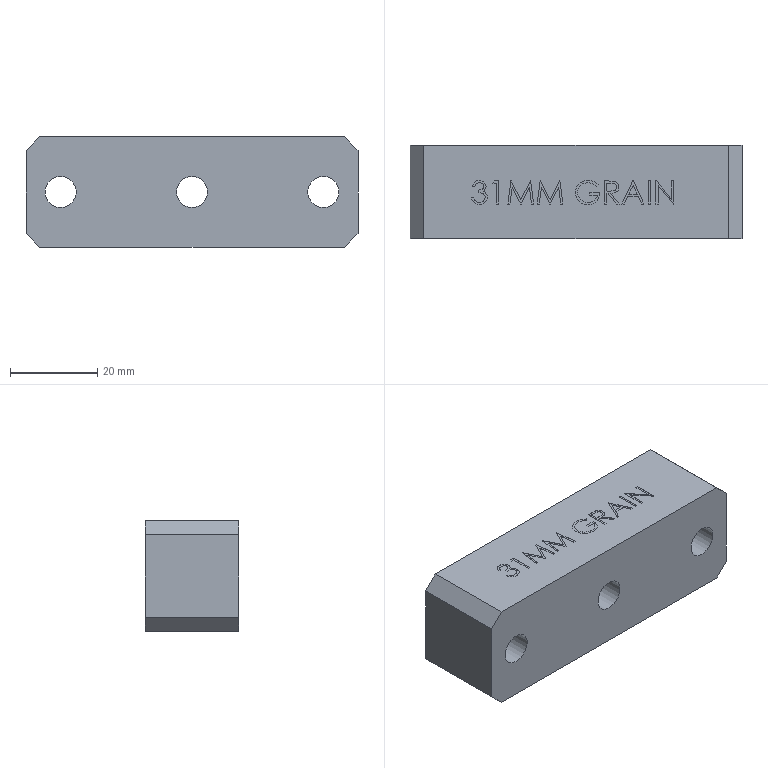CAM job | NX | mm | 3-axis | 2 set-ups | 17 operations | part box 76.2 x 21.43 x 25.4
set-up 1
1. Planar Milling | Mill Mill5 EMC-20A | PLANAR_MILL | path 303.919 mm | 0.1404 min
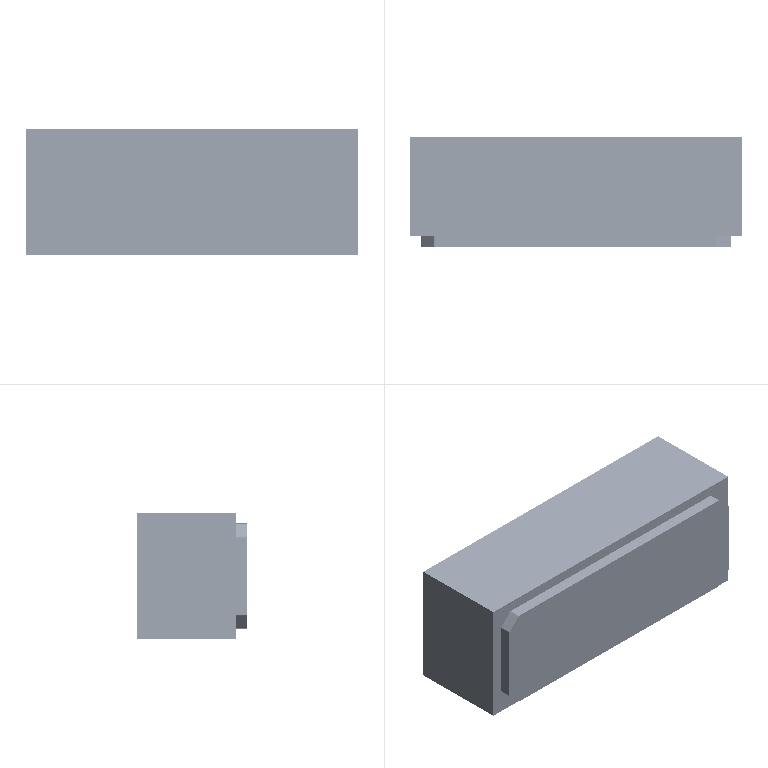2. Face Milling | Mill Mill5 EMC-20A | FACE_MILLING | path 356.465 mm | 0.1677 min
3. Planar Milling | Mill Mill5 2EMC-10A | PLANAR_MILL_1 | path 6144.323 mm | 2.078 min
4. Planar Milling | Mill Mill5 2EMC-10A | PLANAR_MILL_1_COPY | path 6786.153 mm | 2.033 min
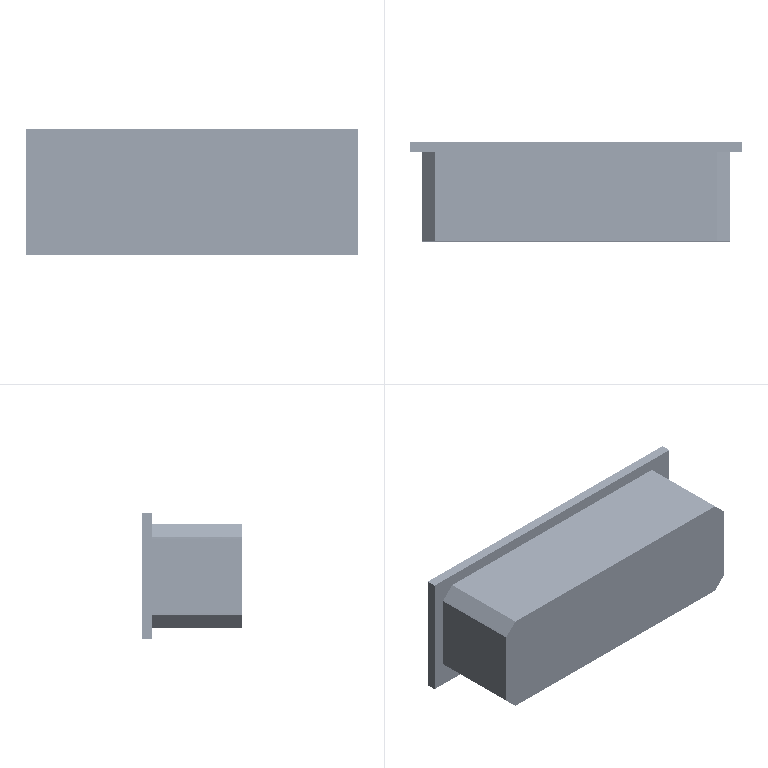5. Point to Point | Drill DrillCenterBell CTR-3-8 | DRILLING | path 104.358 mm | 0.06984 min
6. Point to Point | Drill DrillStandard DR-6.8 | DRILLING_COPY | path 248.616 mm | 0.9937 min
7. Planar Milling | Mill MillChamfer 1CMF-6X90 | PLANAR_MILL_COPY | path 238.379 mm | 0.2338 min
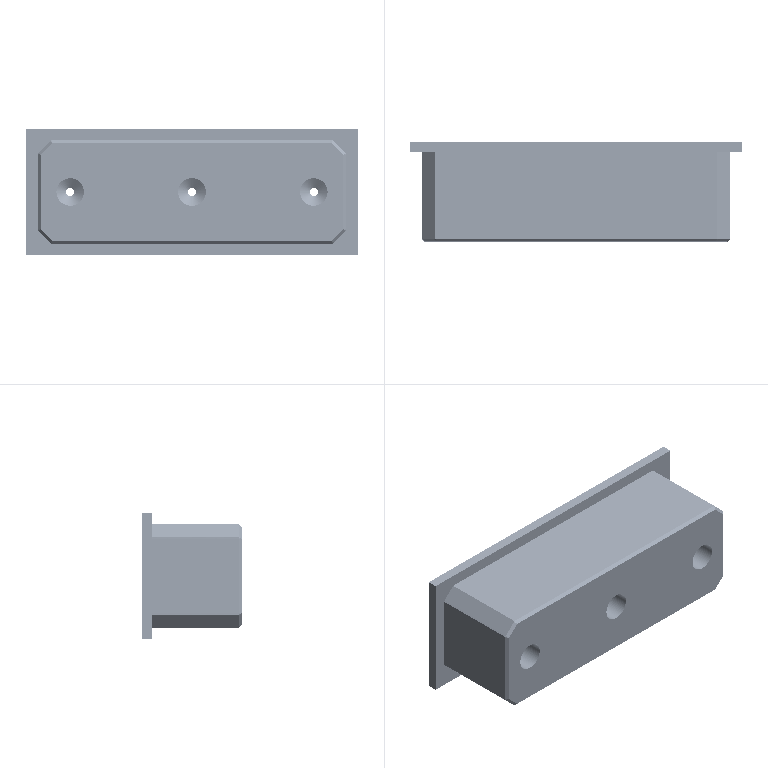8. Planar Milling | Mill MillChamfer 1CMF-6X90 | PLANAR_MILL_COPY_COPY | path 216.811 mm | 0.08832 min
9. Cylinder Milling | Mill Mill5 9EMC-6E | HOLE_MILLING_COPY | path 390.995 mm | 0.7966 min
10. Face Milling | Mill Mill5 8EMC-10E | FACE_MILLING_COPY | path 398.37 mm | 0.5325 min
11. Planar Milling | Mill Mill5 8EMC-10E | PLANAR_MILL_COPY_1 | path 539.578 mm | 0.6883 min
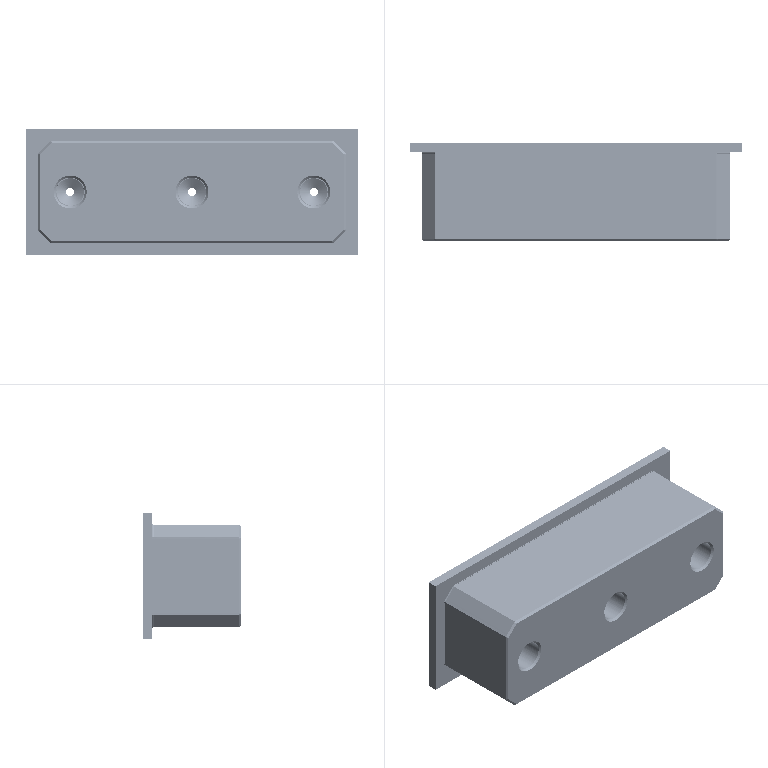12. Planar Milling | Mill MillChamfer 1CMF-6X90 | PLANAR_MILL_COPY_COPY_1 | path 238.379 mm | 0.2338 min
13. Planar Milling | Mill MillChamfer 1CMF-6X90 | PLANAR_MILL_COPY_COPY_COPY | path 216.811 mm | 0.08832 min
set-up 2
14. Face Milling | Mill Mill5 EMC-20A | FACE_MILLING_COPY_1 | path 5809.626 mm | 2.242 min
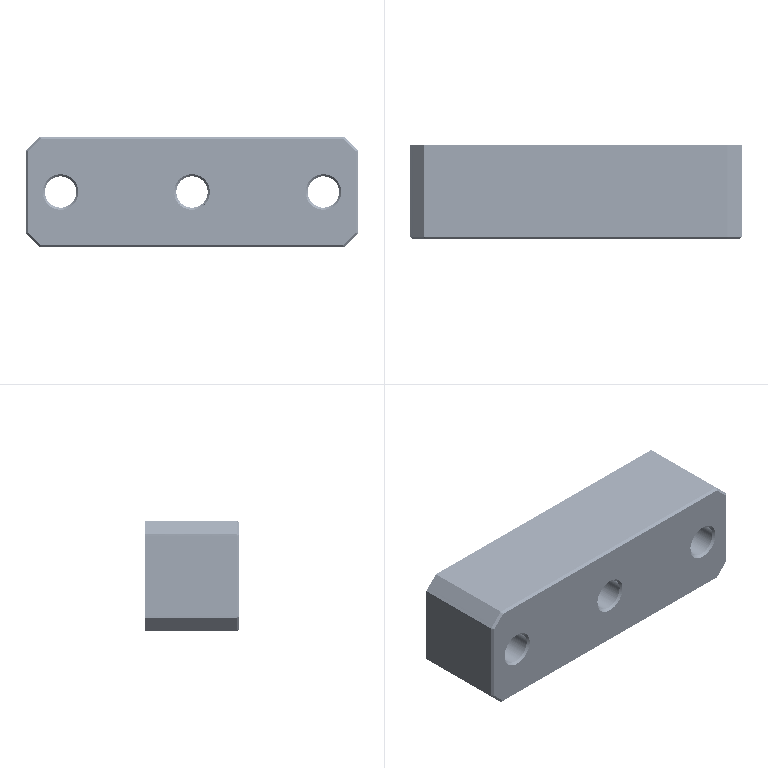15. Face Milling | Mill Mill5 8EMC-10E | FACE_MILLING_COPY_1_COPY | path 404.242 mm | 0.5386 min
16. Planar Milling | Mill MillChamfer 1CMF-6X90 | PLANAR_MILL_COPY_COPY_1_COPY | path 445.057 mm | 0.4637 min
17. Planar Milling | Mill MillChamfer 1CMF-6X90 | PLANAR_MILLING_17 | path 277.851 mm | 0.156 min